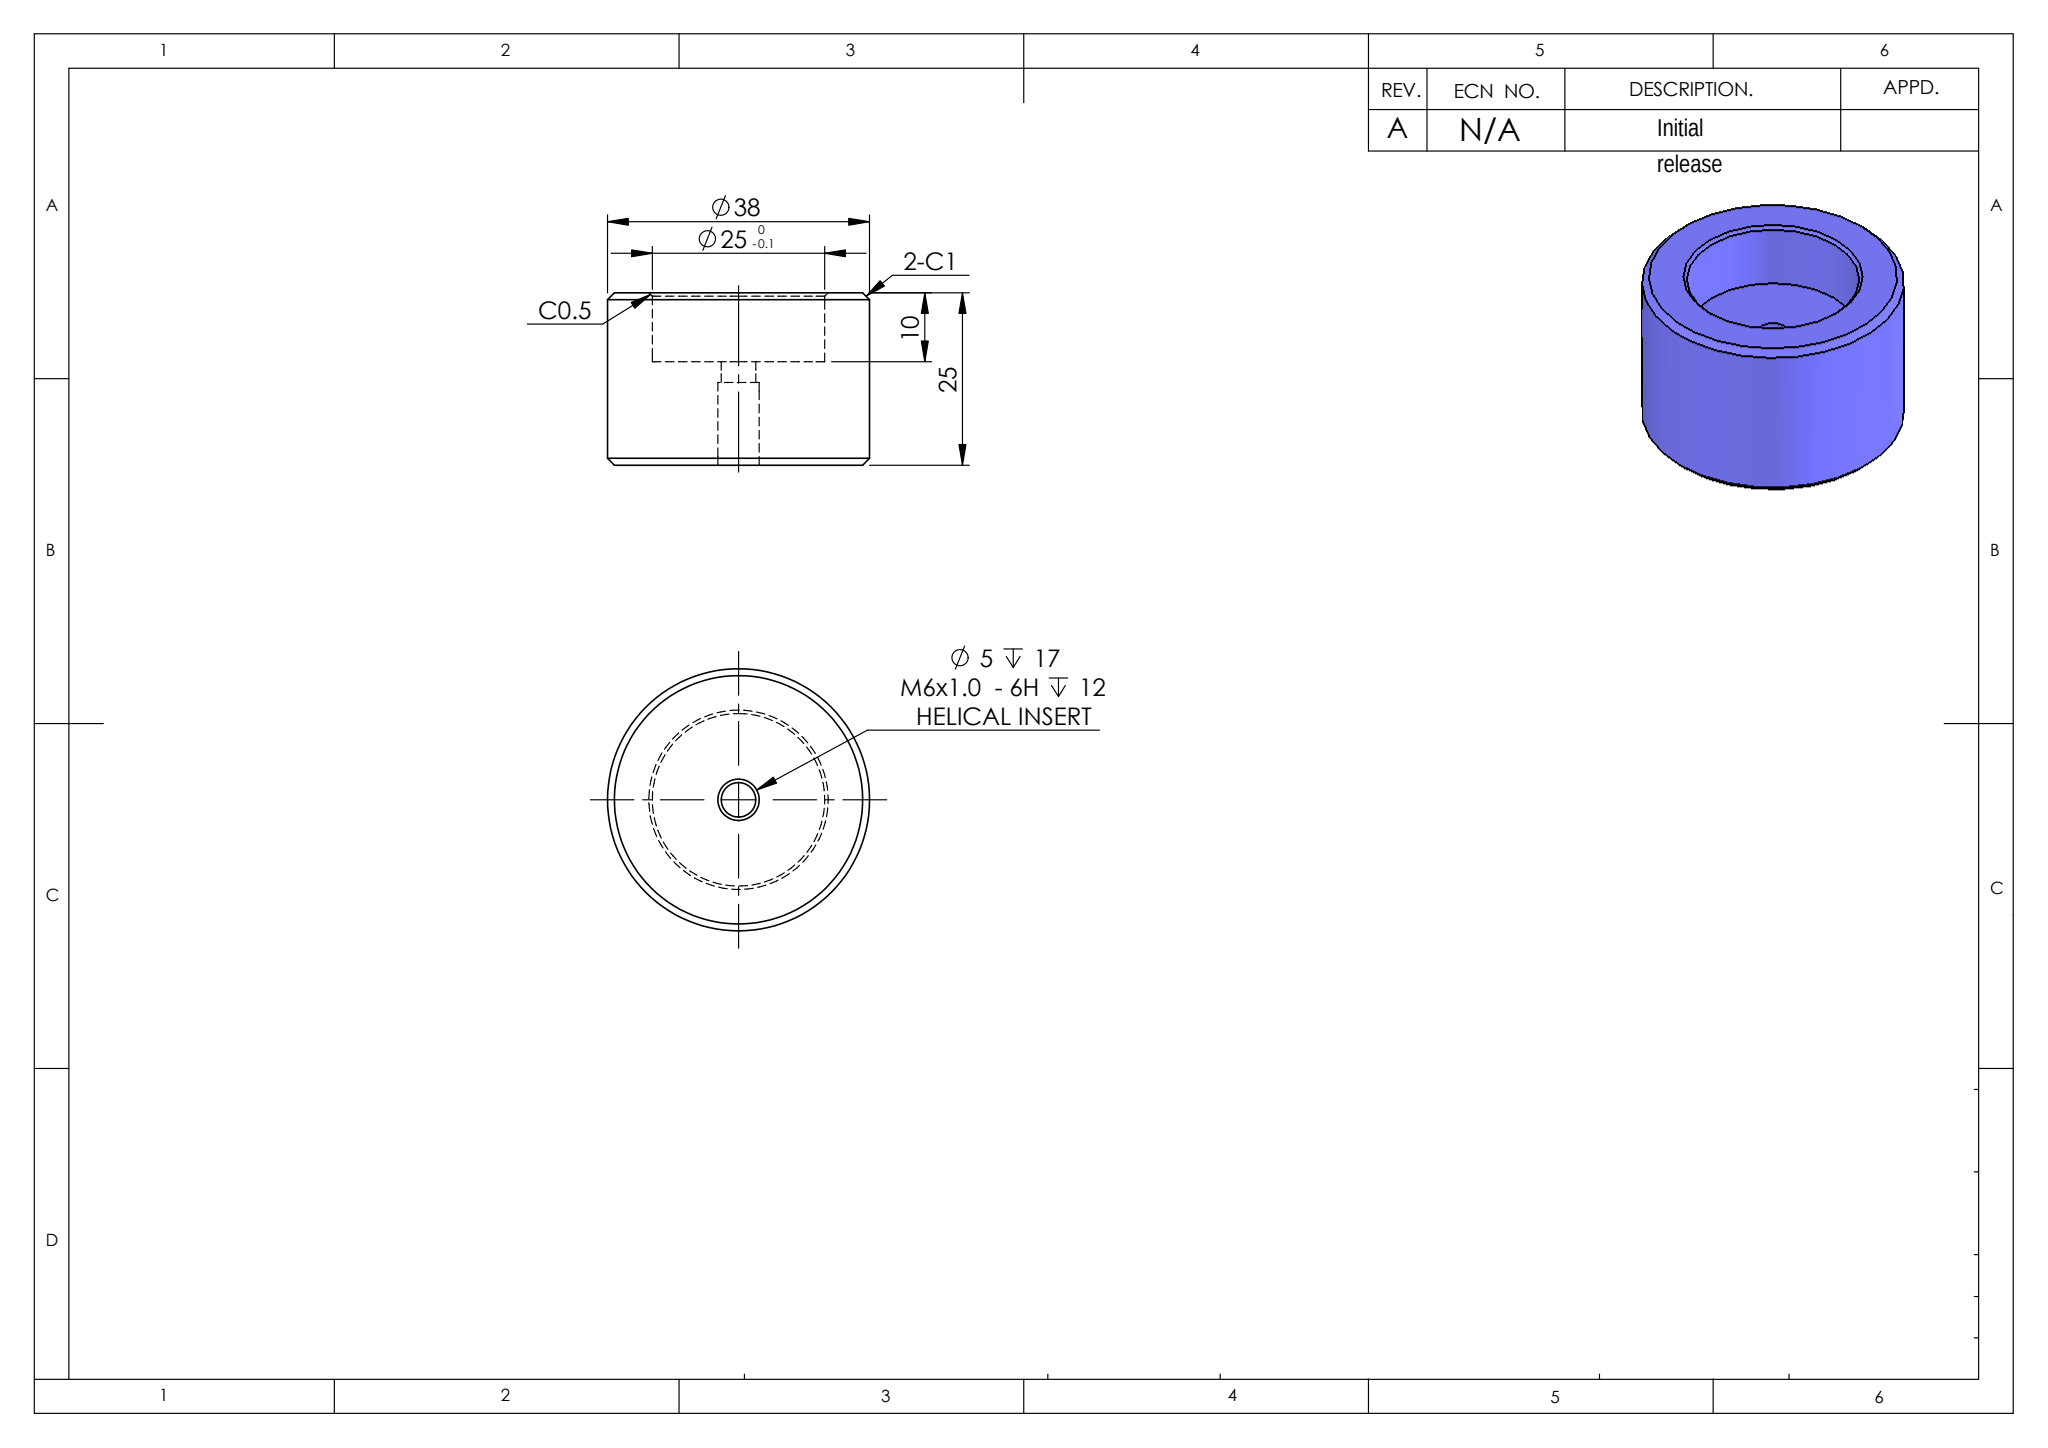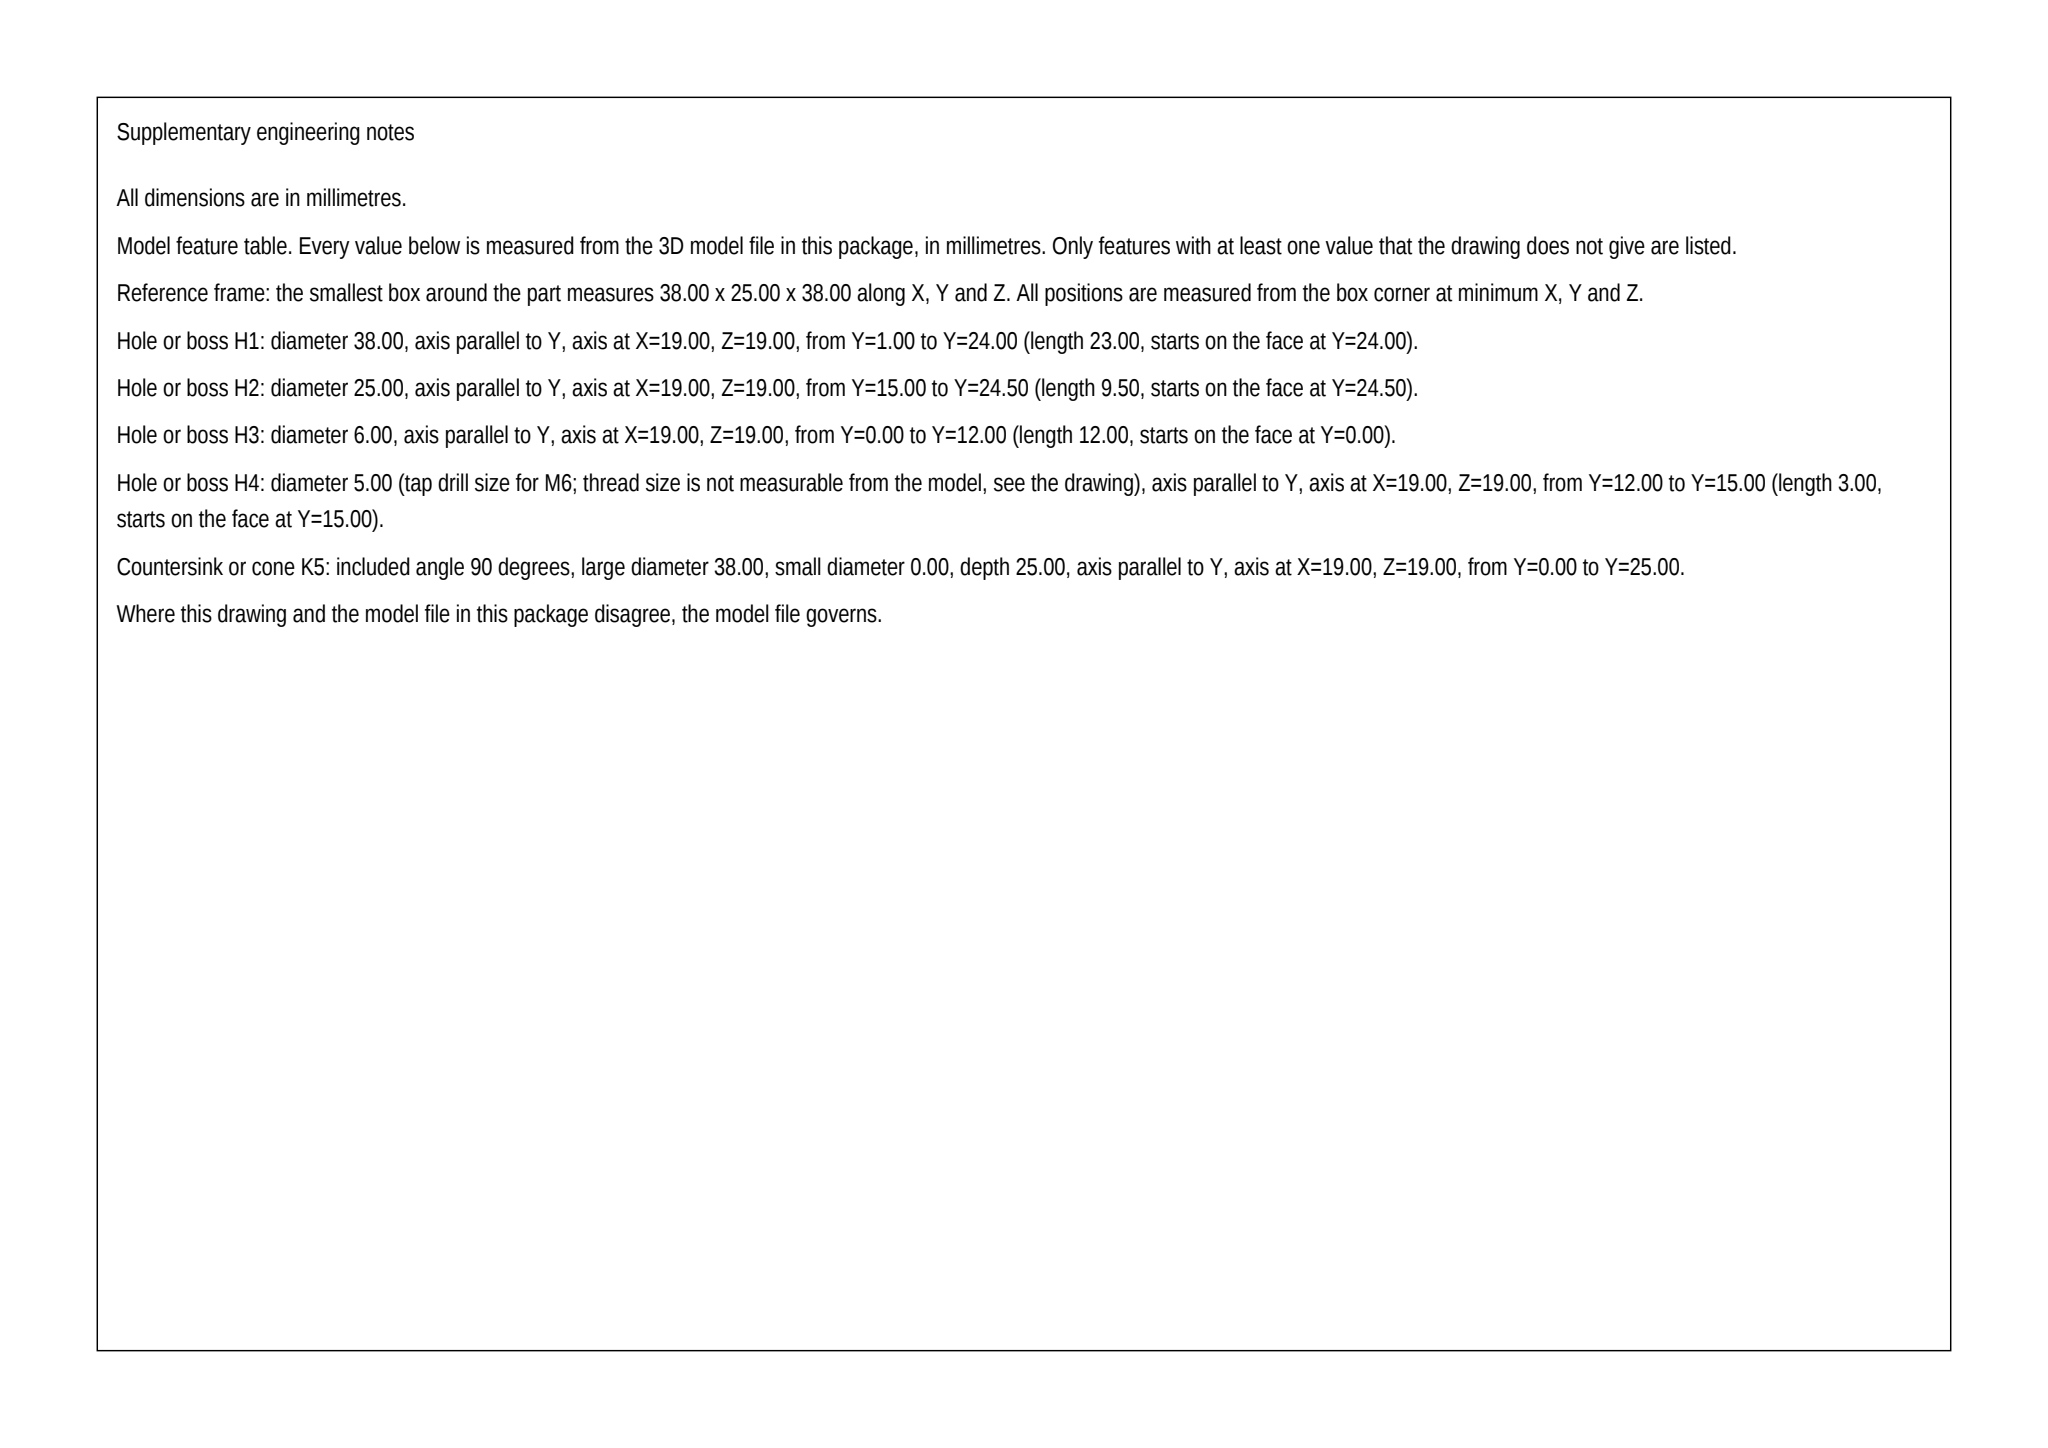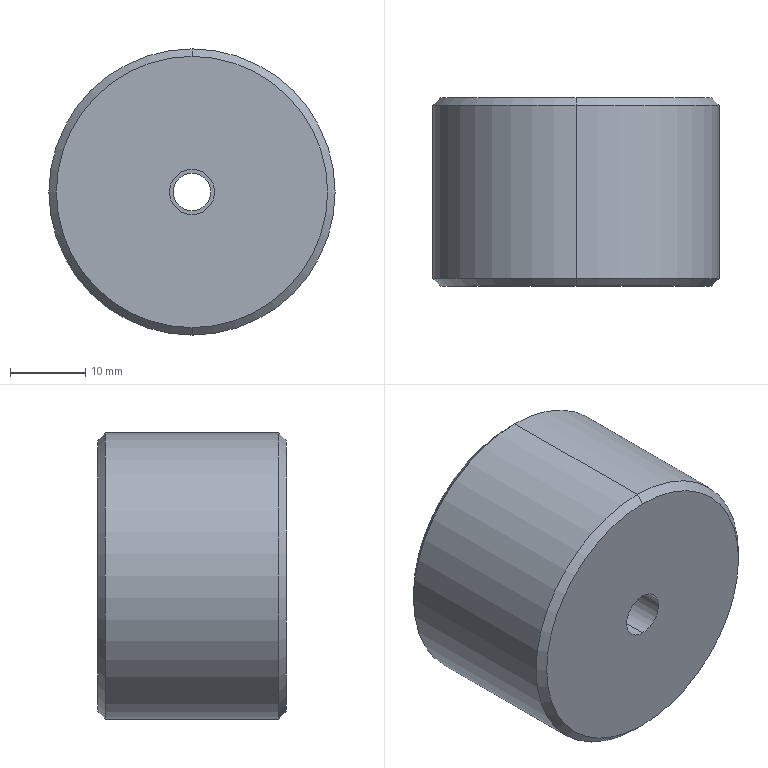Part | SolidWorks | mm | 1 solid | 18 faces | box 38 x 25 x 38 mm | volume 22919 mm3 | cylinder 8 | cone 6 | plane 4 | commonest cylinder face diameters 5 x2 6 x2 25 x2 38 x2
build123d program:
from build123d import *

# Parameters (mm, degrees)
S2D0002_R                   = 19
EXTRUDE1_DEPTH              = 25
SKETCH3_R                   = 12.5
CUT_EXTRUDE1_DEPTH          = 10
M6_TAPPED_HOLE1_D           = 5
M6_TAPPED_HOLE1_DEPTH       = 17
M6_TAPPED_HOLE1_CBORE_D     = 6
M6_TAPPED_HOLE1_CBORE_DEPTH = 12
M6_TAPPED_HOLE1_TIP         = 1.502
CHAMFER1_SIZE               = 1
CHAMFER2_SIZE               = 0.5


with BuildPart() as part:
    # S2D0002 → Extrude1 (new body)
    with BuildSketch(Plane(origin=(0, 0, 0), x_dir=(1, 0, 0), z_dir=(0, 1, 0))):
        with Locations(Location((0, 0, 0), (0, 0, 270))):
            Circle(S2D0002_R)
    extrude(amount=EXTRUDE1_DEPTH)

    # Sketch3 → Cut-Extrude1 (cut)
    with BuildSketch(Plane(origin=(0, 25, 0), x_dir=(-1, 0, 0), z_dir=(0, 1, 0))):
        with Locations(Location((0, 0, 0), (0, 0, 90))):
            Circle(SKETCH3_R)
    extrude(amount=-CUT_EXTRUDE1_DEPTH, mode=Mode.SUBTRACT)

    # M6 Tapped Hole1
    with Locations(Plane.XZ):
        with Locations((0, 0)):
            CounterBoreHole(M6_TAPPED_HOLE1_D / 2, M6_TAPPED_HOLE1_CBORE_D / 2, M6_TAPPED_HOLE1_CBORE_DEPTH, depth=M6_TAPPED_HOLE1_DEPTH)
            with Locations((0, 0, -(M6_TAPPED_HOLE1_DEPTH + M6_TAPPED_HOLE1_TIP / 2))):  # 118° drill point
                Cone(0, M6_TAPPED_HOLE1_D / 2, M6_TAPPED_HOLE1_TIP, mode=Mode.SUBTRACT)

    # Chamfer1
    chamfer1_edges = [part.edges().sort_by_distance(p)[0] for p in [
        (0, 0, -19),
        (0, 25, -19),
    ]]
    chamfer(chamfer1_edges, length=CHAMFER1_SIZE)

    # Chamfer2
    chamfer2_edges = [part.edges().sort_by_distance(p)[0] for p in [
        (0, 25, -12.5),
    ]]
    chamfer(chamfer2_edges, length=CHAMFER2_SIZE)


solid = part.part
STEP:
#1=CARTESIAN_POINT('',(0.,24.5,-12.5));
#2=VERTEX_POINT('',#1);
#3=CARTESIAN_POINT('',(-0.,24.5,12.5));
#4=VERTEX_POINT('',#3);
#5=CARTESIAN_POINT('',(0.,24.5,0.));
#6=DIRECTION('',(0.,1.,0.));
#7=DIRECTION('',(-0.,0.,1.));
#8=AXIS2_PLACEMENT_3D('',#5,#6,#7);
#9=CIRCLE('',#8,12.5);
#10=EDGE_CURVE('',#2,#4,#9,.T.);
#11=ORIENTED_EDGE('',*,*,#10,.F.);
#12=CARTESIAN_POINT('',(0.,25.,-13.));
#13=VERTEX_POINT('',#12);
#14=CARTESIAN_POINT('',(0.,24.5,-12.5));
#15=DIRECTION('',(0.,0.7071,-0.7071));
#16=VECTOR('',#15,1000.);
#17=LINE('',#14,#16);
#18=EDGE_CURVE('',#2,#13,#17,.T.);
#19=ORIENTED_EDGE('',*,*,#18,.T.);
#20=CARTESIAN_POINT('',(-0.,25.,13.));
#21=VERTEX_POINT('',#20);
#22=CARTESIAN_POINT('',(0.,25.,0.));
#23=DIRECTION('',(0.,-1.,0.));
#24=DIRECTION('',(-0.,0.,1.));
#25=AXIS2_PLACEMENT_3D('',#22,#23,#24);
#26=CIRCLE('',#25,13.);
#27=EDGE_CURVE('',#21,#13,#26,.T.);
#28=ORIENTED_EDGE('',*,*,#27,.F.);
#29=CARTESIAN_POINT('',(-0.,24.5,12.5));
#30=DIRECTION('',(-0.,0.7071,0.7071));
#31=VECTOR('',#30,1000.);
#32=LINE('',#29,#31);
#33=EDGE_CURVE('',#4,#21,#32,.T.);
#34=ORIENTED_EDGE('',*,*,#33,.F.);
#35=EDGE_LOOP('',(#11,#19,#28,#34));
#36=FACE_OUTER_BOUND('',#35,.T.);
#37=CARTESIAN_POINT('',(0.,24.5,0.));
#38=DIRECTION('',(0.,1.,0.));
#39=DIRECTION('',(-0.,0.,1.));
#40=AXIS2_PLACEMENT_3D('',#37,#38,#39);
#41=CONICAL_SURFACE('',#40,12.5,0.7854);
#42=ADVANCED_FACE('',(#36),#41,.F.);
#43=CARTESIAN_POINT('',(0.,0.,-18.));
#44=VERTEX_POINT('',#43);
#45=CARTESIAN_POINT('',(-0.,0.,18.));
#46=VERTEX_POINT('',#45);
#47=CARTESIAN_POINT('',(0.,0.,0.));
#48=DIRECTION('',(0.,-1.,0.));
#49=DIRECTION('',(-0.,0.,1.));
#50=AXIS2_PLACEMENT_3D('',#47,#48,#49);
#51=CIRCLE('',#50,18.);
#52=EDGE_CURVE('',#44,#46,#51,.T.);
#53=ORIENTED_EDGE('',*,*,#52,.F.);
#54=CARTESIAN_POINT('',(0.,1.,-19.));
#55=VERTEX_POINT('',#54);
#56=CARTESIAN_POINT('',(0.,1.,-19.));
#57=DIRECTION('',(0.,0.7071,-0.7071));
#58=VECTOR('',#57,1000.);
#59=LINE('',#56,#58);
#60=EDGE_CURVE('',#44,#55,#59,.T.);
#61=ORIENTED_EDGE('',*,*,#60,.T.);
#62=CARTESIAN_POINT('',(0.,1.,19.));
#63=VERTEX_POINT('',#62);
#64=CARTESIAN_POINT('',(0.,1.,0.));
#65=DIRECTION('',(0.,1.,0.));
#66=DIRECTION('',(-0.,0.,1.));
#67=AXIS2_PLACEMENT_3D('',#64,#65,#66);
#68=CIRCLE('',#67,19.);
#69=EDGE_CURVE('',#63,#55,#68,.T.);
#70=ORIENTED_EDGE('',*,*,#69,.F.);
#71=CARTESIAN_POINT('',(-0.,1.,19.));
#72=DIRECTION('',(-0.,0.7071,0.7071));
#73=VECTOR('',#72,1000.);
#74=LINE('',#71,#73);
#75=EDGE_CURVE('',#46,#63,#74,.T.);
#76=ORIENTED_EDGE('',*,*,#75,.F.);
#77=EDGE_LOOP('',(#53,#61,#70,#76));
#78=FACE_OUTER_BOUND('',#77,.T.);
#79=CARTESIAN_POINT('',(0.,1.,0.));
#80=DIRECTION('',(0.,1.,0.));
#81=DIRECTION('',(-0.,0.,1.));
#82=AXIS2_PLACEMENT_3D('',#79,#80,#81);
#83=CONICAL_SURFACE('',#82,19.,0.7854);
#84=ADVANCED_FACE('',(#78),#83,.T.);
#85=CARTESIAN_POINT('',(0.,25.,18.));
#86=VERTEX_POINT('',#85);
#87=CARTESIAN_POINT('',(0.,25.,-18.));
#88=VERTEX_POINT('',#87);
#89=CARTESIAN_POINT('',(0.,25.,0.));
#90=DIRECTION('',(0.,1.,0.));
#91=DIRECTION('',(-0.,0.,1.));
#92=AXIS2_PLACEMENT_3D('',#89,#90,#91);
#93=CIRCLE('',#92,18.);
#94=EDGE_CURVE('',#86,#88,#93,.T.);
#95=ORIENTED_EDGE('',*,*,#94,.F.);
#96=CARTESIAN_POINT('',(0.,24.,19.));
#97=VERTEX_POINT('',#96);
#98=CARTESIAN_POINT('',(0.,25.,18.));
#99=DIRECTION('',(0.,-0.7071,0.7071));
#100=VECTOR('',#99,1000.);
#101=LINE('',#98,#100);
#102=EDGE_CURVE('',#86,#97,#101,.T.);
#103=ORIENTED_EDGE('',*,*,#102,.T.);
#104=CARTESIAN_POINT('',(0.,24.,-19.));
#105=VERTEX_POINT('',#104);
#106=CARTESIAN_POINT('',(0.,24.,0.));
#107=DIRECTION('',(0.,-1.,0.));
#108=DIRECTION('',(-0.,0.,1.));
#109=AXIS2_PLACEMENT_3D('',#106,#107,#108);
#110=CIRCLE('',#109,19.);
#111=EDGE_CURVE('',#105,#97,#110,.T.);
#112=ORIENTED_EDGE('',*,*,#111,.F.);
#113=CARTESIAN_POINT('',(0.,25.,-18.));
#114=DIRECTION('',(0.,-0.7071,-0.7071));
#115=VECTOR('',#114,1000.);
#116=LINE('',#113,#115);
#117=EDGE_CURVE('',#88,#105,#116,.T.);
#118=ORIENTED_EDGE('',*,*,#117,.F.);
#119=EDGE_LOOP('',(#95,#103,#112,#118));
#120=FACE_OUTER_BOUND('',#119,.T.);
#121=CARTESIAN_POINT('',(0.,25.,0.));
#122=DIRECTION('',(0.,-1.,0.));
#123=DIRECTION('',(0.,0.,-1.));
#124=AXIS2_PLACEMENT_3D('',#121,#122,#123);
#125=CONICAL_SURFACE('',#124,18.,0.7854);
#126=ADVANCED_FACE('',(#120),#125,.T.);
#127=CARTESIAN_POINT('',(0.,15.,-2.5));
#128=VERTEX_POINT('',#127);
#129=CARTESIAN_POINT('',(0.,15.,2.5));
#130=VERTEX_POINT('',#129);
#131=CARTESIAN_POINT('',(0.,15.,0.));
#132=DIRECTION('',(0.,1.,0.));
#133=DIRECTION('',(-0.,0.,1.));
#134=AXIS2_PLACEMENT_3D('',#131,#132,#133);
#135=CIRCLE('',#134,2.5);
#136=EDGE_CURVE('',#128,#130,#135,.T.);
#137=ORIENTED_EDGE('',*,*,#136,.T.);
#138=CARTESIAN_POINT('',(0.,12.,2.5));
#139=VERTEX_POINT('',#138);
#140=CARTESIAN_POINT('',(0.,0.,2.5));
#141=DIRECTION('',(0.,-1.,0.));
#142=VECTOR('',#141,1000.);
#143=LINE('',#140,#142);
#144=EDGE_CURVE('',#130,#139,#143,.T.);
#145=ORIENTED_EDGE('',*,*,#144,.T.);
#146=CARTESIAN_POINT('',(0.,12.,-2.5));
#147=VERTEX_POINT('',#146);
#148=CARTESIAN_POINT('',(0.,12.,0.));
#149=DIRECTION('',(0.,-1.,0.));
#150=DIRECTION('',(0.,0.,-1.));
#151=AXIS2_PLACEMENT_3D('',#148,#149,#150);
#152=CIRCLE('',#151,2.5);
#153=EDGE_CURVE('',#139,#147,#152,.T.);
#154=ORIENTED_EDGE('',*,*,#153,.T.);
#155=CARTESIAN_POINT('',(0.,0.,-2.5));
#156=DIRECTION('',(0.,-1.,0.));
#157=VECTOR('',#156,1000.);
#158=LINE('',#155,#157);
#159=EDGE_CURVE('',#128,#147,#158,.T.);
#160=ORIENTED_EDGE('',*,*,#159,.F.);
#161=EDGE_LOOP('',(#137,#145,#154,#160));
#162=FACE_OUTER_BOUND('',#161,.T.);
#163=CARTESIAN_POINT('',(0.,0.,0.));
#164=DIRECTION('',(0.,-1.,0.));
#165=DIRECTION('',(0.,0.,-1.));
#166=AXIS2_PLACEMENT_3D('',#163,#164,#165);
#167=CYLINDRICAL_SURFACE('',#166,2.5);
#168=ADVANCED_FACE('',(#162),#167,.F.);
#169=CARTESIAN_POINT('',(0.,12.,3.));
#170=VERTEX_POINT('',#169);
#171=CARTESIAN_POINT('',(0.,12.,-3.));
#172=VERTEX_POINT('',#171);
#173=CARTESIAN_POINT('',(0.,12.,0.));
#174=DIRECTION('',(0.,-1.,0.));
#175=DIRECTION('',(0.,0.,-1.));
#176=AXIS2_PLACEMENT_3D('',#173,#174,#175);
#177=CIRCLE('',#176,3.);
#178=EDGE_CURVE('',#170,#172,#177,.T.);
#179=ORIENTED_EDGE('',*,*,#178,.F.);
#180=CARTESIAN_POINT('',(0.,0.,3.));
#181=VERTEX_POINT('',#180);
#182=CARTESIAN_POINT('',(0.,0.,3.));
#183=DIRECTION('',(0.,-1.,0.));
#184=VECTOR('',#183,1000.);
#185=LINE('',#182,#184);
#186=EDGE_CURVE('',#170,#181,#185,.T.);
#187=ORIENTED_EDGE('',*,*,#186,.T.);
#188=CARTESIAN_POINT('',(0.,0.,-3.));
#189=VERTEX_POINT('',#188);
#190=CARTESIAN_POINT('',(0.,0.,0.));
#191=DIRECTION('',(0.,-1.,0.));
#192=DIRECTION('',(0.,0.,-1.));
#193=AXIS2_PLACEMENT_3D('',#190,#191,#192);
#194=CIRCLE('',#193,3.);
#195=EDGE_CURVE('',#181,#189,#194,.T.);
#196=ORIENTED_EDGE('',*,*,#195,.T.);
#197=CARTESIAN_POINT('',(0.,0.,-3.));
#198=DIRECTION('',(0.,-1.,0.));
#199=VECTOR('',#198,1000.);
#200=LINE('',#197,#199);
#201=EDGE_CURVE('',#172,#189,#200,.T.);
#202=ORIENTED_EDGE('',*,*,#201,.F.);
#203=EDGE_LOOP('',(#179,#187,#196,#202));
#204=FACE_OUTER_BOUND('',#203,.T.);
#205=CARTESIAN_POINT('',(0.,0.,0.));
#206=DIRECTION('',(0.,-1.,0.));
#207=DIRECTION('',(0.,0.,-1.));
#208=AXIS2_PLACEMENT_3D('',#205,#206,#207);
#209=CYLINDRICAL_SURFACE('',#208,3.);
#210=ADVANCED_FACE('',(#204),#209,.F.);
#211=CARTESIAN_POINT('',(0.,15.,-12.5));
#212=VERTEX_POINT('',#211);
#213=CARTESIAN_POINT('',(-0.,15.,12.5));
#214=VERTEX_POINT('',#213);
#215=CARTESIAN_POINT('',(0.,15.,0.));
#216=DIRECTION('',(0.,1.,0.));
#217=DIRECTION('',(-0.,0.,1.));
#218=AXIS2_PLACEMENT_3D('',#215,#216,#217);
#219=CIRCLE('',#218,12.5);
#220=EDGE_CURVE('',#212,#214,#219,.T.);
#221=ORIENTED_EDGE('',*,*,#220,.F.);
#222=CARTESIAN_POINT('',(0.,15.,-12.5));
#223=DIRECTION('',(0.,1.,0.));
#224=VECTOR('',#223,1000.);
#225=LINE('',#222,#224);
#226=EDGE_CURVE('',#212,#2,#225,.T.);
#227=ORIENTED_EDGE('',*,*,#226,.T.);
#228=ORIENTED_EDGE('',*,*,#10,.T.);
#229=CARTESIAN_POINT('',(-0.,15.,12.5));
#230=DIRECTION('',(0.,1.,0.));
#231=VECTOR('',#230,1000.);
#232=LINE('',#229,#231);
#233=EDGE_CURVE('',#214,#4,#232,.T.);
#234=ORIENTED_EDGE('',*,*,#233,.F.);
#235=EDGE_LOOP('',(#221,#227,#228,#234));
#236=FACE_OUTER_BOUND('',#235,.T.);
#237=CARTESIAN_POINT('',(0.,15.,0.));
#238=DIRECTION('',(0.,1.,0.));
#239=DIRECTION('',(-0.,0.,1.));
#240=AXIS2_PLACEMENT_3D('',#237,#238,#239);
#241=CYLINDRICAL_SURFACE('',#240,12.5);
#242=ADVANCED_FACE('',(#236),#241,.F.);
#243=ORIENTED_EDGE('',*,*,#111,.T.);
#244=CARTESIAN_POINT('',(0.,25.,19.));
#245=DIRECTION('',(0.,-1.,0.));
#246=VECTOR('',#245,1000.);
#247=LINE('',#244,#246);
#248=EDGE_CURVE('',#97,#63,#247,.T.);
#249=ORIENTED_EDGE('',*,*,#248,.T.);
#250=ORIENTED_EDGE('',*,*,#69,.T.);
#251=CARTESIAN_POINT('',(0.,25.,-19.));
#252=DIRECTION('',(0.,-1.,0.));
#253=VECTOR('',#252,1000.);
#254=LINE('',#251,#253);
#255=EDGE_CURVE('',#105,#55,#254,.T.);
#256=ORIENTED_EDGE('',*,*,#255,.F.);
#257=EDGE_LOOP('',(#243,#249,#250,#256));
#258=FACE_OUTER_BOUND('',#257,.T.);
#259=CARTESIAN_POINT('',(0.,25.,0.));
#260=DIRECTION('',(0.,-1.,0.));
#261=DIRECTION('',(0.,0.,-1.));
#262=AXIS2_PLACEMENT_3D('',#259,#260,#261);
#263=CYLINDRICAL_SURFACE('',#262,19.);
#264=ADVANCED_FACE('',(#258),#263,.T.);
#265=ORIENTED_EDGE('',*,*,#248,.F.);
#266=CARTESIAN_POINT('',(0.,24.,0.));
#267=DIRECTION('',(0.,-1.,0.));
#268=DIRECTION('',(-0.,0.,1.));
#269=AXIS2_PLACEMENT_3D('',#266,#267,#268);
#270=CIRCLE('',#269,19.);
#271=EDGE_CURVE('',#97,#105,#270,.T.);
#272=ORIENTED_EDGE('',*,*,#271,.T.);
#273=ORIENTED_EDGE('',*,*,#255,.T.);
#274=CARTESIAN_POINT('',(0.,1.,0.));
#275=DIRECTION('',(0.,1.,0.));
#276=DIRECTION('',(-0.,0.,1.));
#277=AXIS2_PLACEMENT_3D('',#274,#275,#276);
#278=CIRCLE('',#277,19.);
#279=EDGE_CURVE('',#55,#63,#278,.T.);
#280=ORIENTED_EDGE('',*,*,#279,.T.);
#281=EDGE_LOOP('',(#265,#272,#273,#280));
#282=FACE_OUTER_BOUND('',#281,.T.);
#283=CARTESIAN_POINT('',(0.,25.,0.));
#284=DIRECTION('',(0.,-1.,0.));
#285=DIRECTION('',(0.,0.,-1.));
#286=AXIS2_PLACEMENT_3D('',#283,#284,#285);
#287=CYLINDRICAL_SURFACE('',#286,19.);
#288=ADVANCED_FACE('',(#282),#287,.T.);
#289=ORIENTED_EDGE('',*,*,#27,.T.);
#290=CARTESIAN_POINT('',(0.,25.,0.));
#291=DIRECTION('',(0.,-1.,0.));
#292=DIRECTION('',(-0.,0.,1.));
#293=AXIS2_PLACEMENT_3D('',#290,#291,#292);
#294=CIRCLE('',#293,13.);
#295=EDGE_CURVE('',#13,#21,#294,.T.);
#296=ORIENTED_EDGE('',*,*,#295,.T.);
#297=EDGE_LOOP('',(#289,#296));
#298=FACE_BOUND('',#297,.T.);
#299=CARTESIAN_POINT('',(0.,25.,0.));
#300=DIRECTION('',(0.,1.,0.));
#301=DIRECTION('',(-0.,0.,1.));
#302=AXIS2_PLACEMENT_3D('',#299,#300,#301);
#303=CIRCLE('',#302,18.);
#304=EDGE_CURVE('',#88,#86,#303,.T.);
#305=ORIENTED_EDGE('',*,*,#304,.T.);
#306=ORIENTED_EDGE('',*,*,#94,.T.);
#307=EDGE_LOOP('',(#305,#306));
#308=FACE_OUTER_BOUND('',#307,.T.);
#309=CARTESIAN_POINT('',(0.,25.,0.));
#310=DIRECTION('',(0.,1.,0.));
#311=DIRECTION('',(-0.,0.,1.));
#312=AXIS2_PLACEMENT_3D('',#309,#310,#311);
#313=PLANE('',#312);
#314=ADVANCED_FACE('',(#298,#308),#313,.T.);
#315=CARTESIAN_POINT('',(0.,0.,0.));
#316=DIRECTION('',(0.,-1.,0.));
#317=DIRECTION('',(-0.,0.,1.));
#318=AXIS2_PLACEMENT_3D('',#315,#316,#317);
#319=CIRCLE('',#318,18.);
#320=EDGE_CURVE('',#46,#44,#319,.T.);
#321=ORIENTED_EDGE('',*,*,#320,.T.);
#322=ORIENTED_EDGE('',*,*,#52,.T.);
#323=EDGE_LOOP('',(#321,#322));
#324=FACE_OUTER_BOUND('',#323,.T.);
#325=CARTESIAN_POINT('',(0.,0.,0.));
#326=DIRECTION('',(0.,-1.,0.));
#327=DIRECTION('',(0.,0.,-1.));
#328=AXIS2_PLACEMENT_3D('',#325,#326,#327);
#329=CIRCLE('',#328,3.);
#330=EDGE_CURVE('',#189,#181,#329,.T.);
#331=ORIENTED_EDGE('',*,*,#330,.F.);
#332=ORIENTED_EDGE('',*,*,#195,.F.);
#333=EDGE_LOOP('',(#331,#332));
#334=FACE_BOUND('',#333,.T.);
#335=CARTESIAN_POINT('',(0.,0.,0.));
#336=DIRECTION('',(0.,1.,0.));
#337=DIRECTION('',(-0.,0.,1.));
#338=AXIS2_PLACEMENT_3D('',#335,#336,#337);
#339=PLANE('',#338);
#340=ADVANCED_FACE('',(#324,#334),#339,.F.);
#341=ORIENTED_EDGE('',*,*,#226,.F.);
#342=CARTESIAN_POINT('',(0.,15.,0.));
#343=DIRECTION('',(0.,1.,0.));
#344=DIRECTION('',(-0.,0.,1.));
#345=AXIS2_PLACEMENT_3D('',#342,#343,#344);
#346=CIRCLE('',#345,12.5);
#347=EDGE_CURVE('',#214,#212,#346,.T.);
#348=ORIENTED_EDGE('',*,*,#347,.F.);
#349=ORIENTED_EDGE('',*,*,#233,.T.);
#350=CARTESIAN_POINT('',(0.,24.5,0.));
#351=DIRECTION('',(0.,1.,0.));
#352=DIRECTION('',(-0.,0.,1.));
#353=AXIS2_PLACEMENT_3D('',#350,#351,#352);
#354=CIRCLE('',#353,12.5);
#355=EDGE_CURVE('',#4,#2,#354,.T.);
#356=ORIENTED_EDGE('',*,*,#355,.T.);
#357=EDGE_LOOP('',(#341,#348,#349,#356));
#358=FACE_OUTER_BOUND('',#357,.T.);
#359=CARTESIAN_POINT('',(0.,15.,0.));
#360=DIRECTION('',(0.,1.,0.));
#361=DIRECTION('',(-0.,0.,1.));
#362=AXIS2_PLACEMENT_3D('',#359,#360,#361);
#363=CYLINDRICAL_SURFACE('',#362,12.5);
#364=ADVANCED_FACE('',(#358),#363,.F.);
#365=ORIENTED_EDGE('',*,*,#136,.F.);
#366=CARTESIAN_POINT('',(0.,15.,0.));
#367=DIRECTION('',(0.,1.,0.));
#368=DIRECTION('',(-0.,0.,1.));
#369=AXIS2_PLACEMENT_3D('',#366,#367,#368);
#370=CIRCLE('',#369,2.5);
#371=EDGE_CURVE('',#130,#128,#370,.T.);
#372=ORIENTED_EDGE('',*,*,#371,.F.);
#373=EDGE_LOOP('',(#365,#372));
#374=FACE_BOUND('',#373,.T.);
#375=ORIENTED_EDGE('',*,*,#347,.T.);
#376=ORIENTED_EDGE('',*,*,#220,.T.);
#377=EDGE_LOOP('',(#375,#376));
#378=FACE_OUTER_BOUND('',#377,.T.);
#379=CARTESIAN_POINT('',(0.,15.,0.));
#380=DIRECTION('',(0.,1.,0.));
#381=DIRECTION('',(-0.,0.,1.));
#382=AXIS2_PLACEMENT_3D('',#379,#380,#381);
#383=PLANE('',#382);
#384=ADVANCED_FACE('',(#374,#378),#383,.T.);
#385=ORIENTED_EDGE('',*,*,#186,.F.);
#386=CARTESIAN_POINT('',(0.,12.,0.));
#387=DIRECTION('',(0.,-1.,0.));
#388=DIRECTION('',(0.,0.,-1.));
#389=AXIS2_PLACEMENT_3D('',#386,#387,#388);
#390=CIRCLE('',#389,3.);
#391=EDGE_CURVE('',#172,#170,#390,.T.);
#392=ORIENTED_EDGE('',*,*,#391,.F.);
#393=ORIENTED_EDGE('',*,*,#201,.T.);
#394=ORIENTED_EDGE('',*,*,#330,.T.);
#395=EDGE_LOOP('',(#385,#392,#393,#394));
#396=FACE_OUTER_BOUND('',#395,.T.);
#397=CARTESIAN_POINT('',(0.,0.,0.));
#398=DIRECTION('',(0.,-1.,0.));
#399=DIRECTION('',(0.,0.,-1.));
#400=AXIS2_PLACEMENT_3D('',#397,#398,#399);
#401=CYLINDRICAL_SURFACE('',#400,3.);
#402=ADVANCED_FACE('',(#396),#401,.F.);
#403=CARTESIAN_POINT('',(0.,12.,0.));
#404=DIRECTION('',(0.,-1.,0.));
#405=DIRECTION('',(0.,0.,-1.));
#406=AXIS2_PLACEMENT_3D('',#403,#404,#405);
#407=CIRCLE('',#406,2.5);
#408=EDGE_CURVE('',#147,#139,#407,.T.);
#409=ORIENTED_EDGE('',*,*,#408,.F.);
#410=ORIENTED_EDGE('',*,*,#153,.F.);
#411=EDGE_LOOP('',(#409,#410));
#412=FACE_BOUND('',#411,.T.);
#413=ORIENTED_EDGE('',*,*,#391,.T.);
#414=ORIENTED_EDGE('',*,*,#178,.T.);
#415=EDGE_LOOP('',(#413,#414));
#416=FACE_OUTER_BOUND('',#415,.T.);
#417=CARTESIAN_POINT('',(2.5,12.,-0.));
#418=DIRECTION('',(0.,1.,0.));
#419=DIRECTION('',(-0.,0.,1.));
#420=AXIS2_PLACEMENT_3D('',#417,#418,#419);
#421=PLANE('',#420);
#422=ADVANCED_FACE('',(#412,#416),#421,.F.);
#423=ORIENTED_EDGE('',*,*,#144,.F.);
#424=ORIENTED_EDGE('',*,*,#371,.T.);
#425=ORIENTED_EDGE('',*,*,#159,.T.);
#426=ORIENTED_EDGE('',*,*,#408,.T.);
#427=EDGE_LOOP('',(#423,#424,#425,#426));
#428=FACE_OUTER_BOUND('',#427,.T.);
#429=CARTESIAN_POINT('',(0.,0.,0.));
#430=DIRECTION('',(0.,-1.,0.));
#431=DIRECTION('',(0.,0.,-1.));
#432=AXIS2_PLACEMENT_3D('',#429,#430,#431);
#433=CYLINDRICAL_SURFACE('',#432,2.5);
#434=ADVANCED_FACE('',(#428),#433,.F.);
#435=ORIENTED_EDGE('',*,*,#102,.F.);
#436=ORIENTED_EDGE('',*,*,#304,.F.);
#437=ORIENTED_EDGE('',*,*,#117,.T.);
#438=ORIENTED_EDGE('',*,*,#271,.F.);
#439=EDGE_LOOP('',(#435,#436,#437,#438));
#440=FACE_OUTER_BOUND('',#439,.T.);
#441=CARTESIAN_POINT('',(0.,25.,0.));
#442=DIRECTION('',(0.,-1.,0.));
#443=DIRECTION('',(0.,0.,-1.));
#444=AXIS2_PLACEMENT_3D('',#441,#442,#443);
#445=CONICAL_SURFACE('',#444,18.,0.7854);
#446=ADVANCED_FACE('',(#440),#445,.T.);
#447=ORIENTED_EDGE('',*,*,#60,.F.);
#448=ORIENTED_EDGE('',*,*,#320,.F.);
#449=ORIENTED_EDGE('',*,*,#75,.T.);
#450=ORIENTED_EDGE('',*,*,#279,.F.);
#451=EDGE_LOOP('',(#447,#448,#449,#450));
#452=FACE_OUTER_BOUND('',#451,.T.);
#453=CARTESIAN_POINT('',(0.,1.,0.));
#454=DIRECTION('',(0.,1.,0.));
#455=DIRECTION('',(-0.,0.,1.));
#456=AXIS2_PLACEMENT_3D('',#453,#454,#455);
#457=CONICAL_SURFACE('',#456,19.,0.7854);
#458=ADVANCED_FACE('',(#452),#457,.T.);
#459=ORIENTED_EDGE('',*,*,#18,.F.);
#460=ORIENTED_EDGE('',*,*,#355,.F.);
#461=ORIENTED_EDGE('',*,*,#33,.T.);
#462=ORIENTED_EDGE('',*,*,#295,.F.);
#463=EDGE_LOOP('',(#459,#460,#461,#462));
#464=FACE_OUTER_BOUND('',#463,.T.);
#465=CARTESIAN_POINT('',(0.,24.5,0.));
#466=DIRECTION('',(0.,1.,0.));
#467=DIRECTION('',(-0.,0.,1.));
#468=AXIS2_PLACEMENT_3D('',#465,#466,#467);
#469=CONICAL_SURFACE('',#468,12.5,0.7854);
#470=ADVANCED_FACE('',(#464),#469,.F.);
#471=CLOSED_SHELL('',(#42,#84,#126,#168,#210,#242,#264,#288,#314,#340,#364,#384,#402,#422,#434,#446,#458,#470));
#472=MANIFOLD_SOLID_BREP('',#471);
#473=CARTESIAN_POINT('',(0.,0.,0.));
#474=DIRECTION('',(0.,0.,1.));
#475=DIRECTION('',(1.,0.,0.));
#476=AXIS2_PLACEMENT_3D('',#473,#474,#475);
#477=(LENGTH_UNIT()NAMED_UNIT(*)SI_UNIT(.MILLI.,.METRE.));
#478=UNCERTAINTY_MEASURE_WITH_UNIT(LENGTH_MEASURE(0.00001),#477,'','');
#479=(NAMED_UNIT(*)PLANE_ANGLE_UNIT()SI_UNIT($,.RADIAN.));
#480=(NAMED_UNIT(*)SI_UNIT($,.STERADIAN.)SOLID_ANGLE_UNIT());
#481=(GEOMETRIC_REPRESENTATION_CONTEXT(3)GLOBAL_UNCERTAINTY_ASSIGNED_CONTEXT((#478))GLOBAL_UNIT_ASSIGNED_CONTEXT((#477,#479,#480))REPRESENTATION_CONTEXT('',''));
#482=ADVANCED_BREP_SHAPE_REPRESENTATION('',(#472,#476),#481);